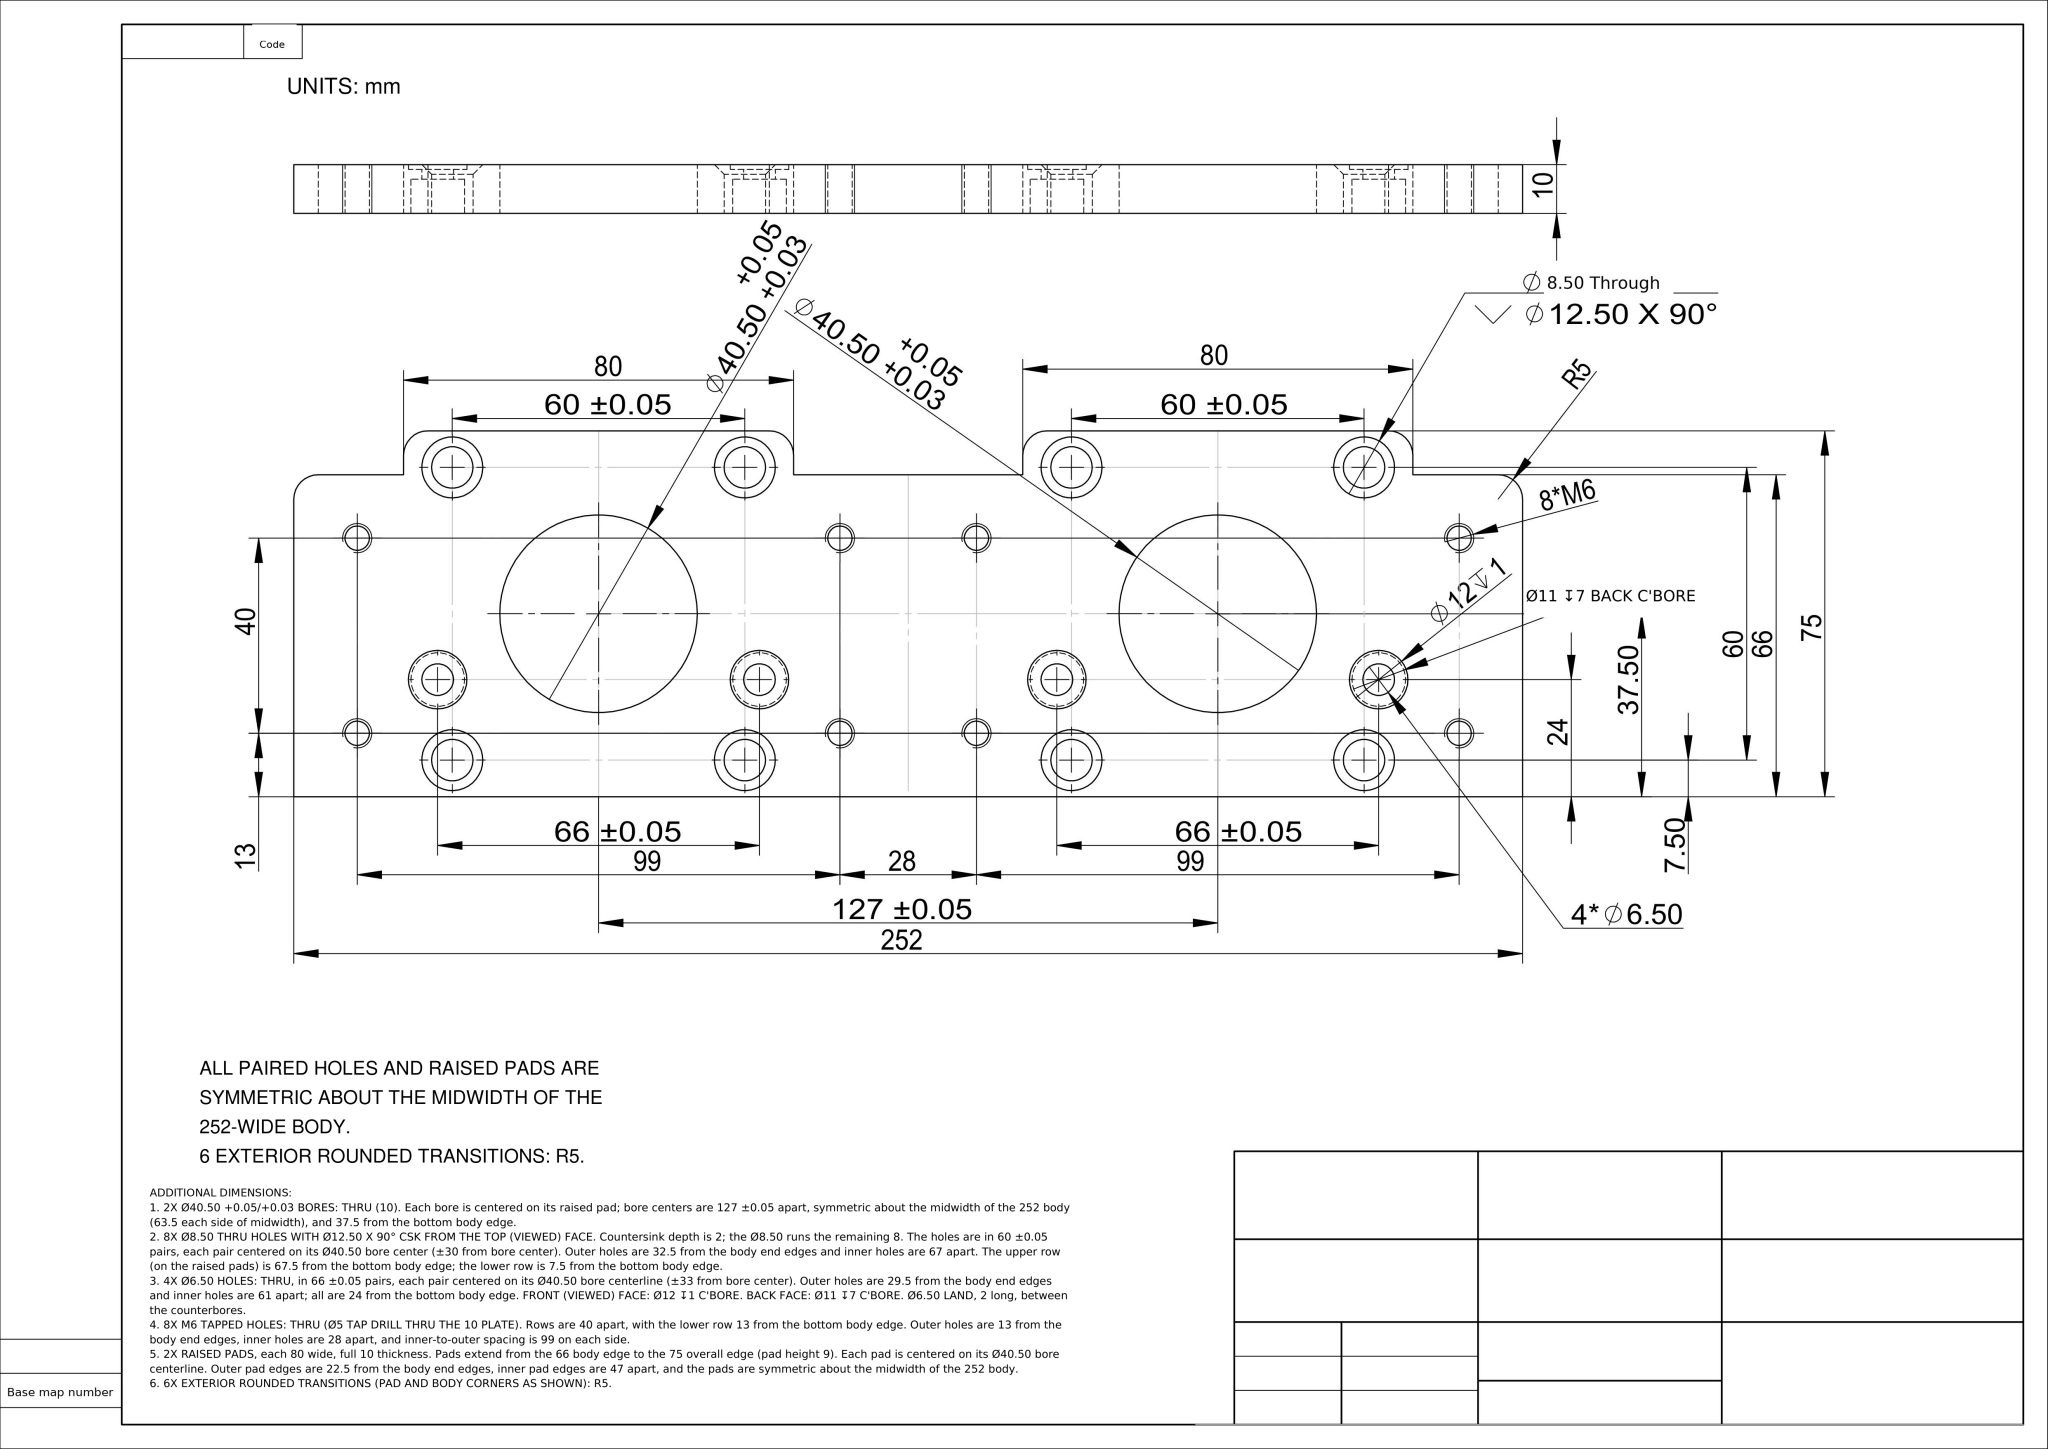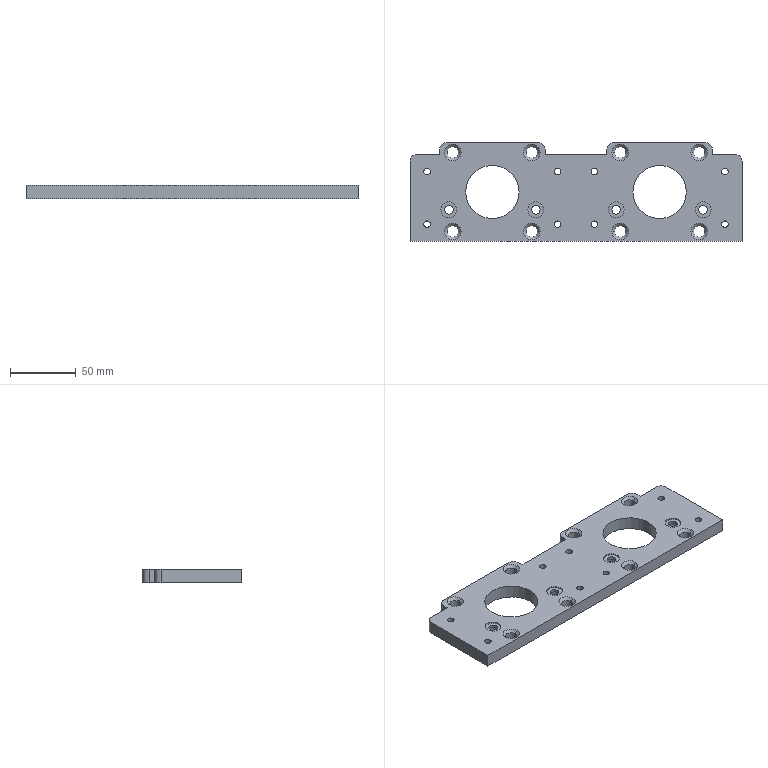Part | NX | mm | 1 solid | 104 faces | box 252 x 75 x 10 mm | volume 144650 mm3 | cylinder 66 | plane 22 | cone 16 | commonest cylinder face diameters 5 x16 8.5 x16 12 x8 11 x8 6.5 x8 10 x6 40.5 x4